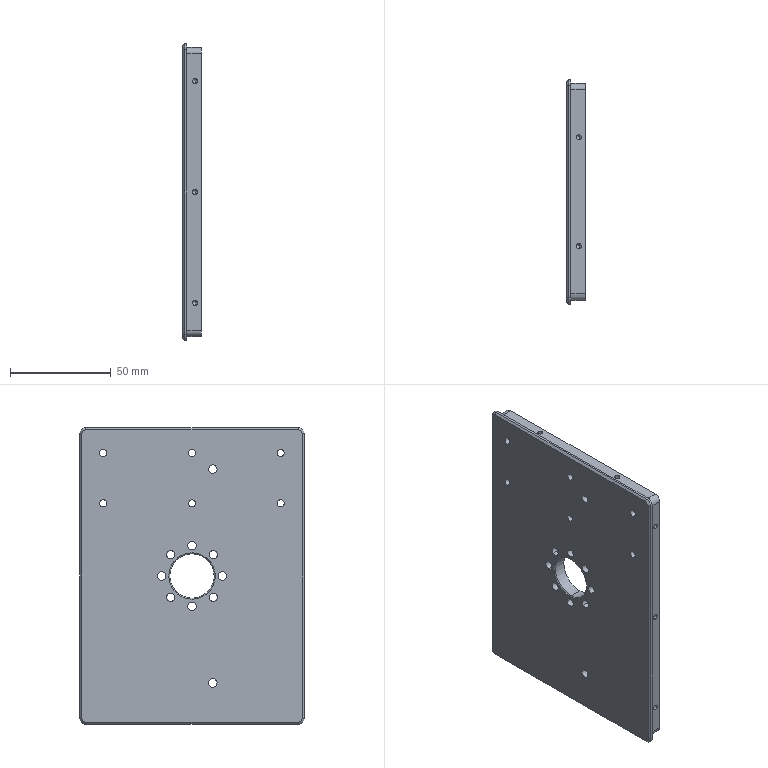CAM job | Mastercam | mm | 16 operations | part box 9 x 111.2 x 147.2
1. Facing | 24 - 100 平铣刀
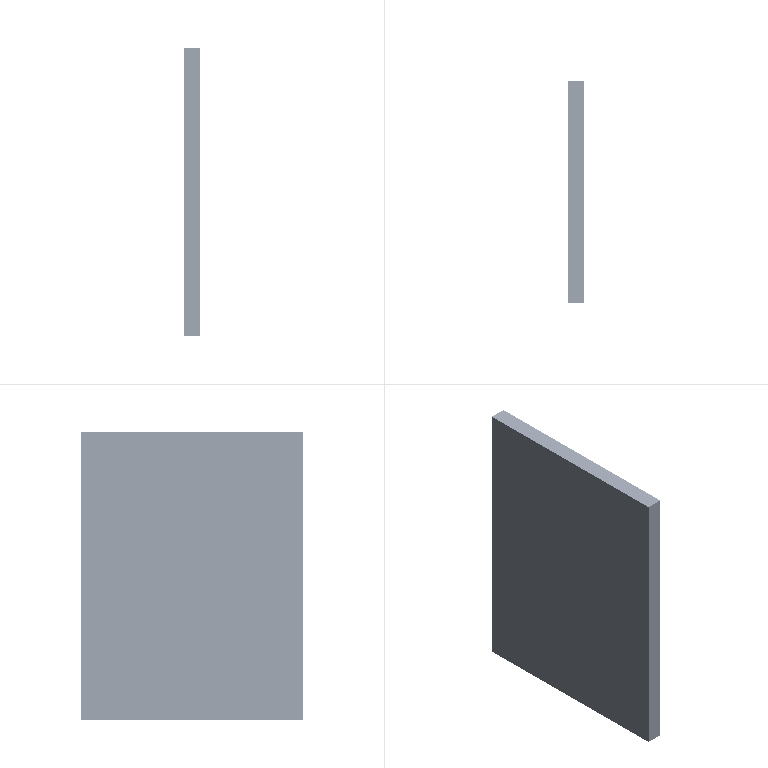2. 2D High Speed (2D Dynamic Mill) | 11 - 12 平铣刀
3. Contour (Ramp) | 11 - 12 平铣刀
4. Contour (Ramp) | 11 - 12 平铣刀
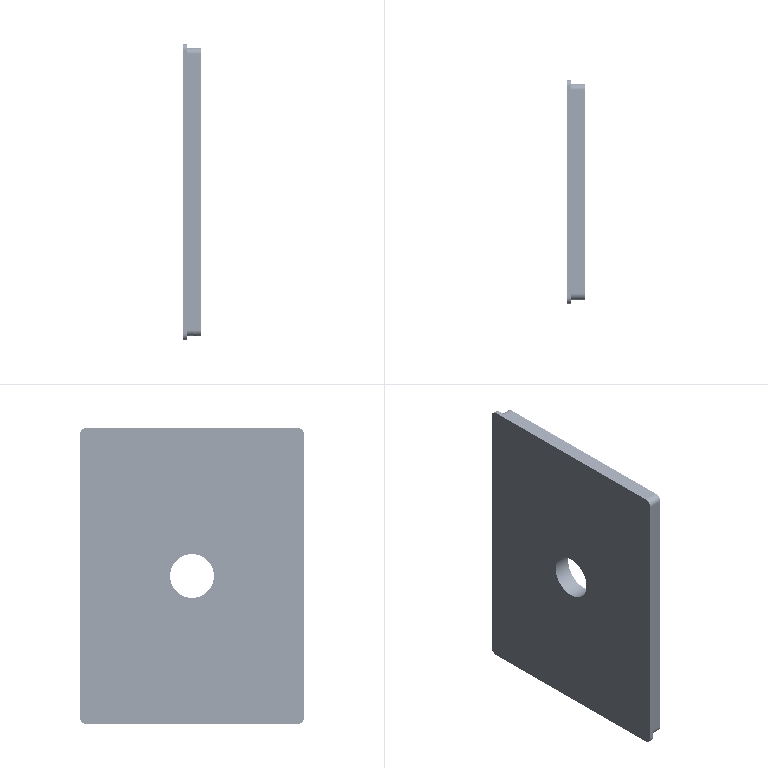5. Contour (Ramp) | 11 - 12 平铣刀
6. Contour (2D) | 12 - 12 平铣刀
7. Contour (2D) | 12 - 12 平铣刀
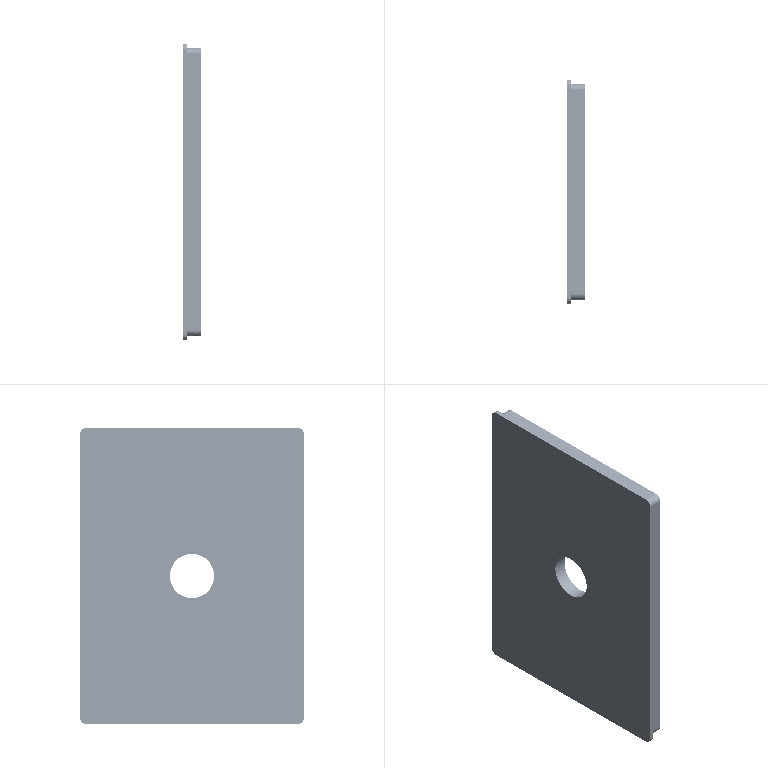8. Contour (2D) | 12 - 12 平铣刀
9. Contour (2D) | 12 - 12 平铣刀
10. Drill/Counterbore | 5 - 4 倒角刀
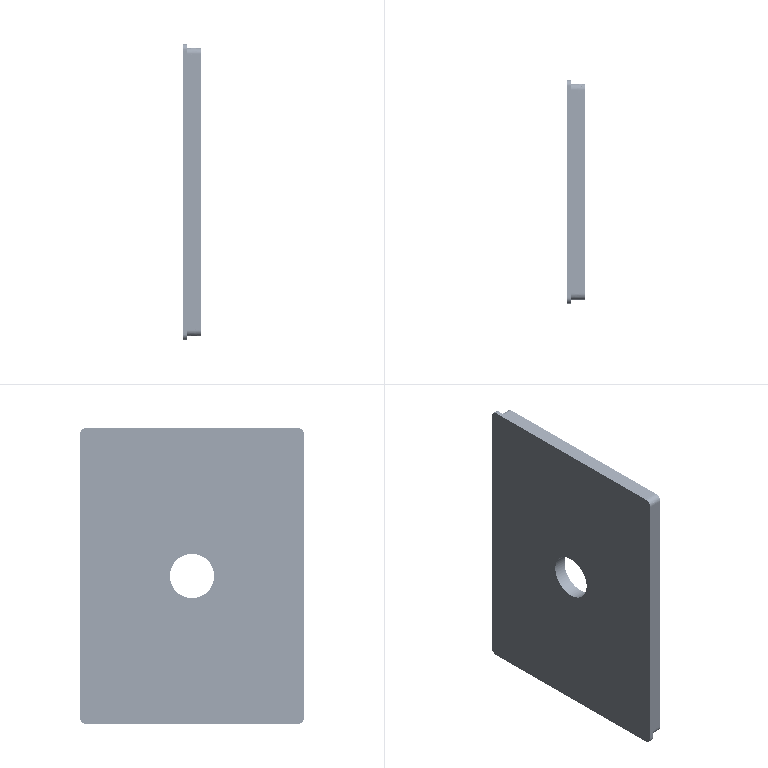11. Contour (2D chamfer) | 5 - 4 倒角刀
12. Facing | 9 - 10 平铣刀
13. Facing | 24 - 100 平铣刀
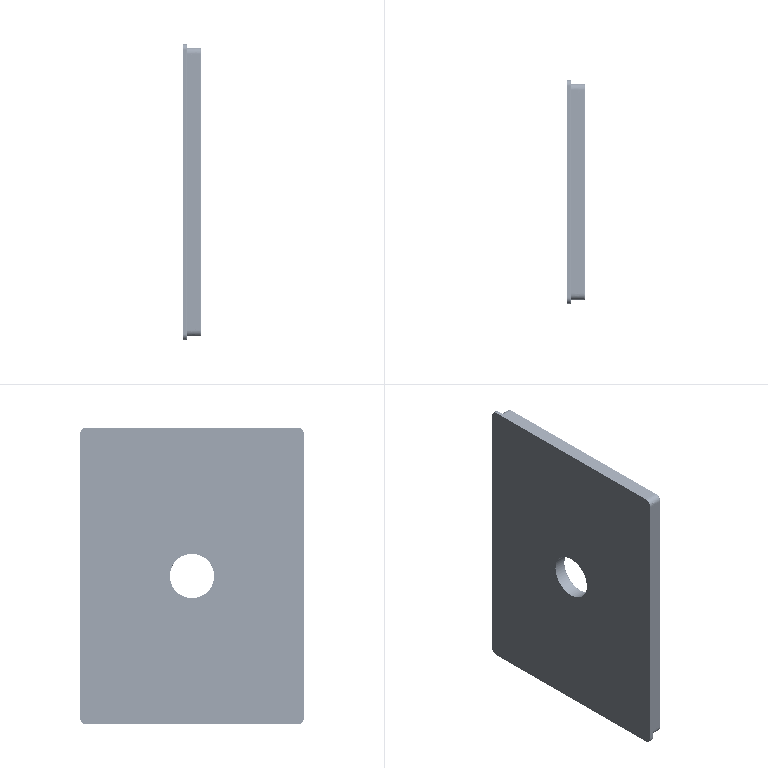14. Contour (2D chamfer) | 7 - 6 倒角刀
15. Drill/Counterbore | 5 - 4 倒角刀
16. Drill/Counterbore | 5 - 4 倒角刀